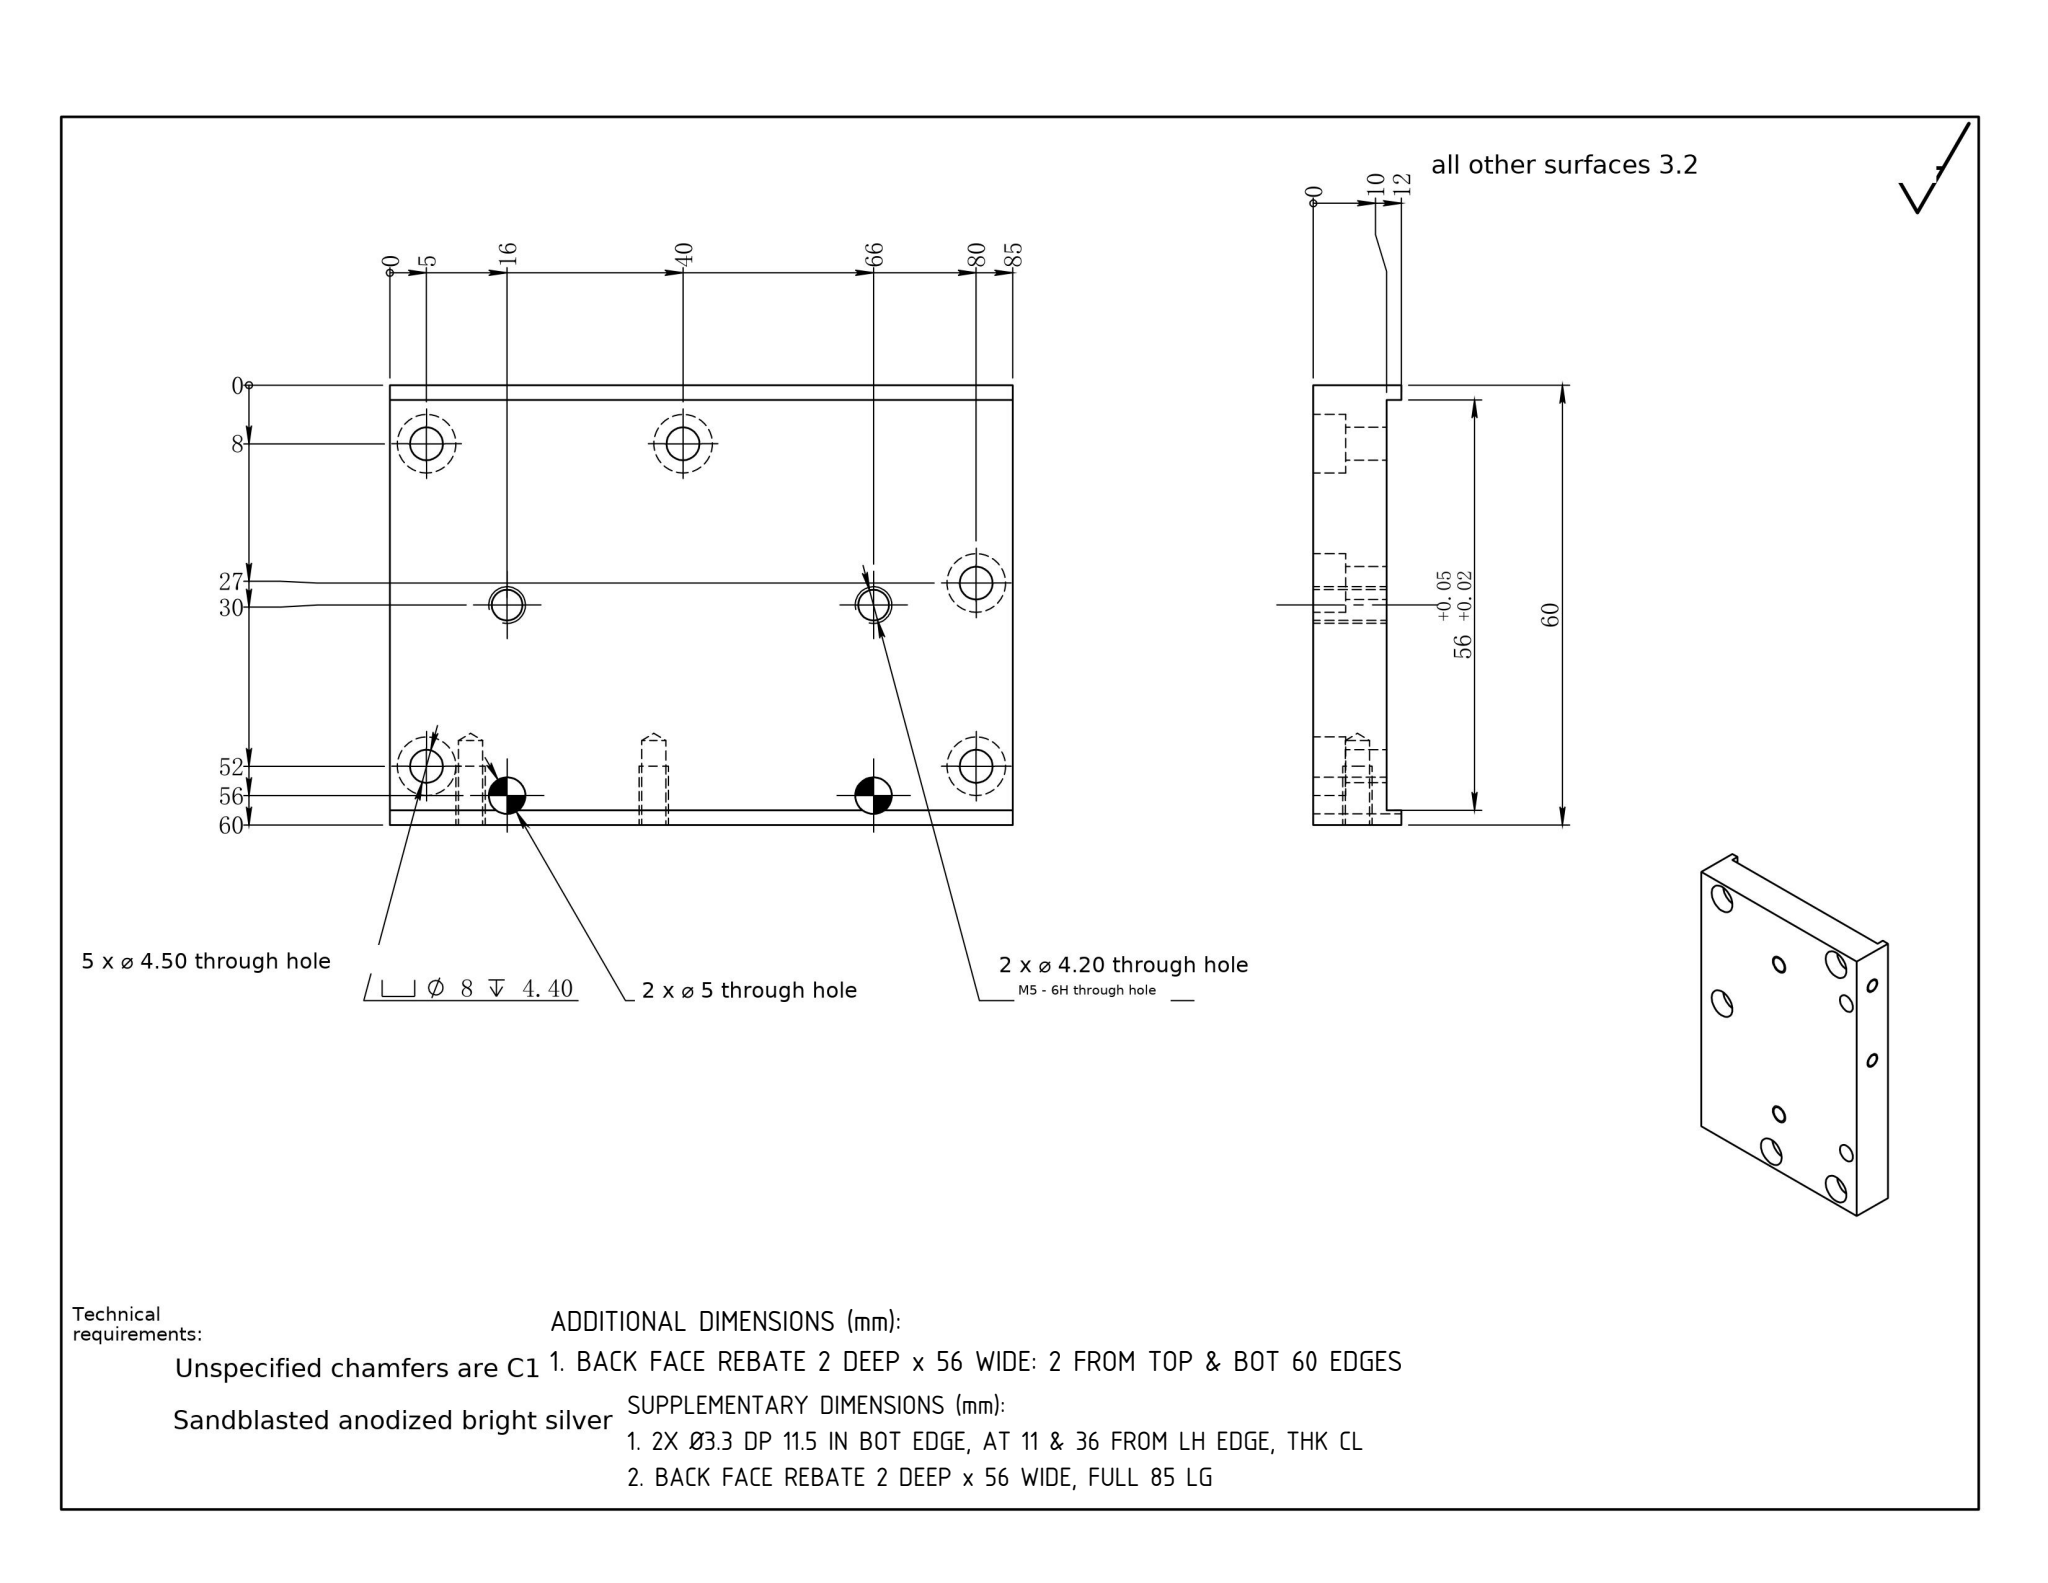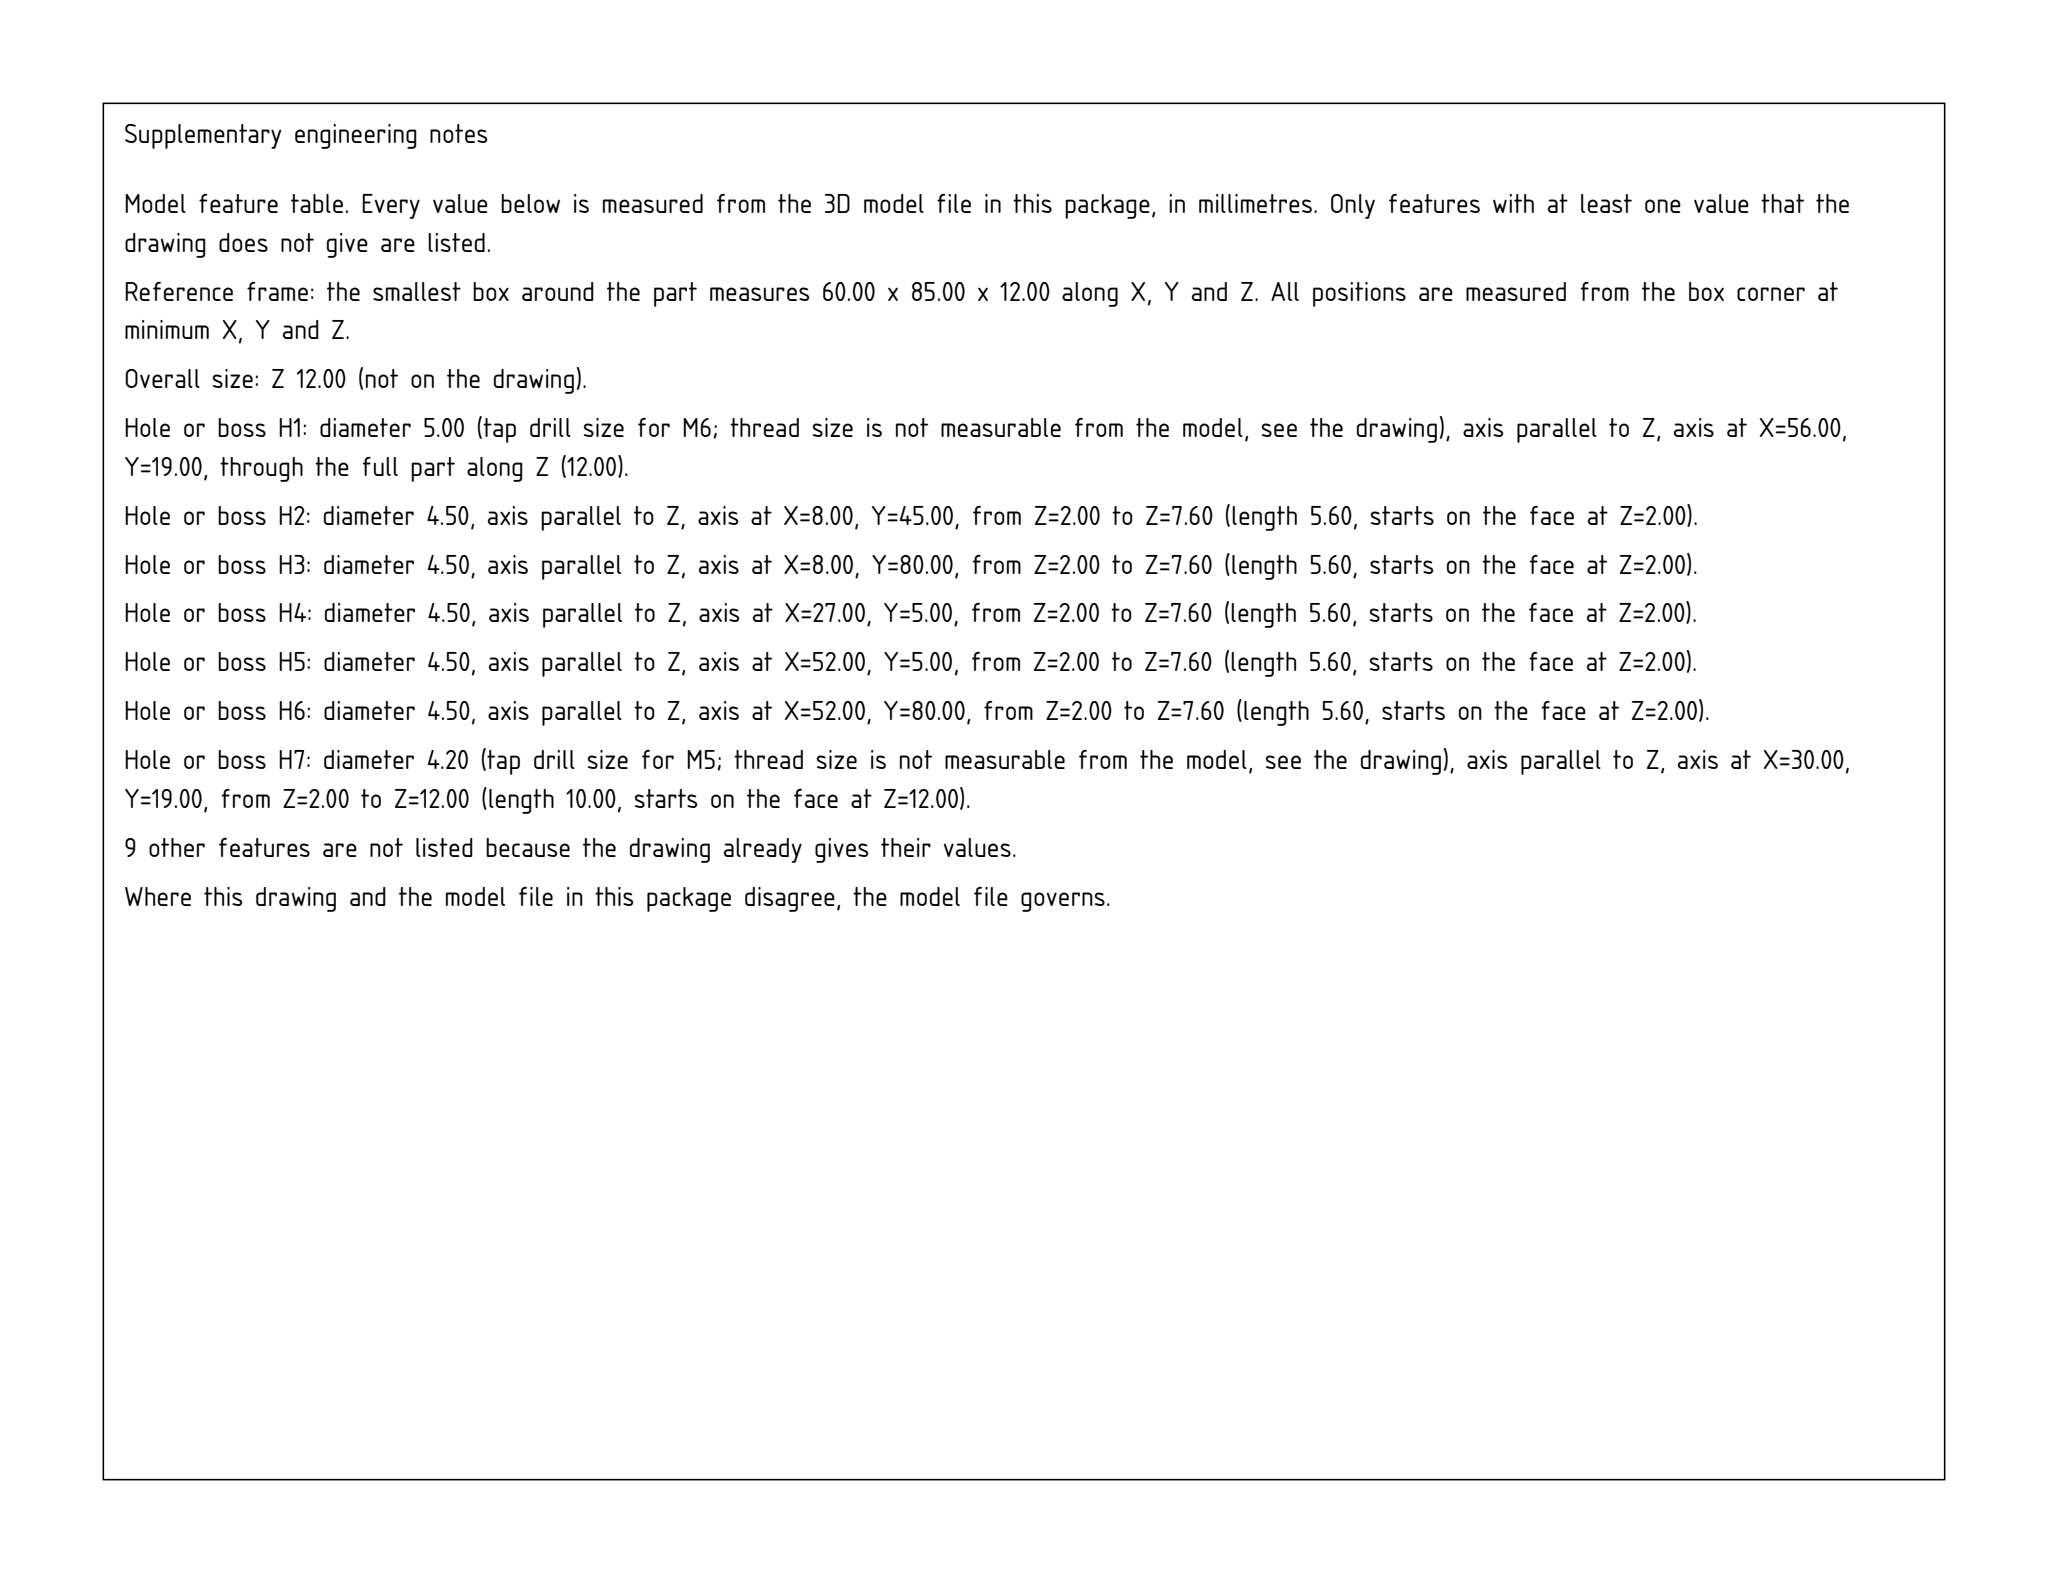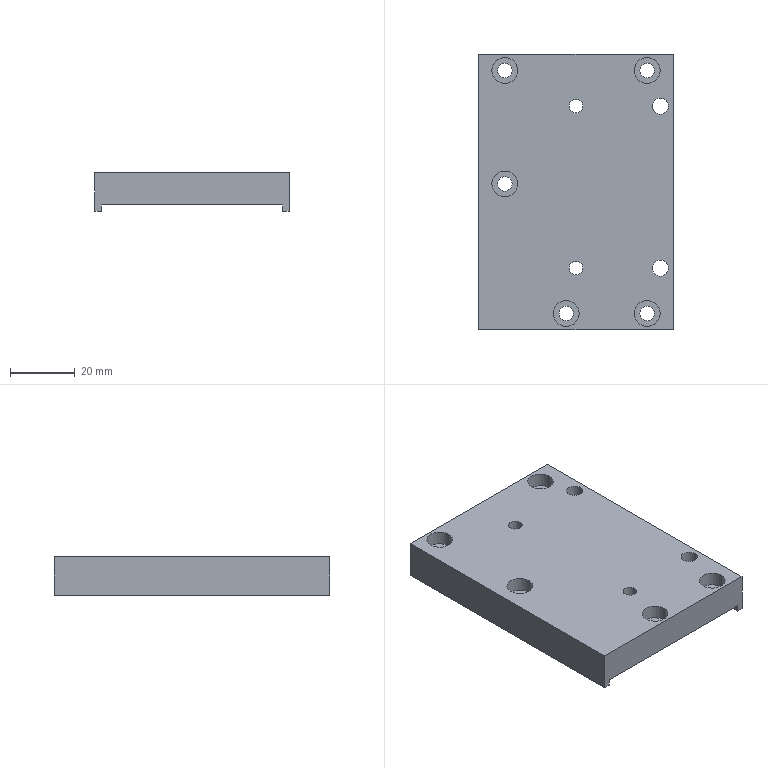Part | SolidWorks | mm | 1 solid | 53 faces | box 60 x 85 x 12 mm | volume 49253 mm3 | cylinder 32 | plane 17 | cone 4 | commonest cylinder face diameters 8 x10 4.5 x10 3.3 x4 5 x4 4.2 x4
build123d program:
from build123d import *

# Parameters (mm, degrees)
SKETCH1_W                                       = 60
SKETCH1_H                                       = 85
BOSS_EXTRUDE1_DEPTH                             = 6
M5_TAPPED_HOLE1_D                               = 4.2
F_5_0_5_DIAMETER_HOLE1_D                        = 5
SKETCH8_W                                       = 56
SKETCH8_H                                       = 85
CUT_EXTRUDE1_DEPTH                              = 2
M4_HEX_SOCKET_HEAD_CAP_SCREW_CBORE1_D           = 4.5
M4_HEX_SOCKET_HEAD_CAP_SCREW_CBORE1_CBORE_D     = 8
M4_HEX_SOCKET_HEAD_CAP_SCREW_CBORE1_CBORE_DEPTH = 4.4
M4_TAPPED_HOLE1_D                               = 3.3
M4_TAPPED_HOLE1_DEPTH                           = 11.5
M4_TAPPED_HOLE1_TIP                             = 0.9914


with BuildPart() as part:
    # Sketch1 → Boss-Extrude1 (new, symmetric)
    with BuildSketch(Plane.XY):
        Rectangle(SKETCH1_W, SKETCH1_H)
    extrude(amount=BOSS_EXTRUDE1_DEPTH, both=True)

    # M5 Tapped Hole1 (through all)
    with Locations(Plane.XY.offset(6)):
        with Locations((0, -23.5), (0, 26.5)):
            Hole(M5_TAPPED_HOLE1_D / 2)

    # 5.0 _5_ Diameter Hole1 (through all)
    with Locations(Plane(origin=(0, 0, -6), x_dir=(-1, 0, 0), z_dir=(0, 0, -1))):
        with Locations((-26, -23.5), (-26, 26.5)):
            Hole(F_5_0_5_DIAMETER_HOLE1_D / 2)

    # Sketch8 → Cut-Extrude1 (cut)
    with BuildSketch(Plane(origin=(0, 0, -6), x_dir=(-1, 0, 0), z_dir=(0, 0, -1))):
        Rectangle(SKETCH8_W, SKETCH8_H)
    extrude(amount=-CUT_EXTRUDE1_DEPTH, mode=Mode.SUBTRACT)

    # M4 Hex Socket Head Cap Screw CBORE1 (through all)
    with Locations(Plane.XY.offset(6)):
        with Locations((-22, 37.5), (22, 37.5), (-22, 2.5), (-3, -37.5), (22, -37.5)):
            CounterBoreHole(M4_HEX_SOCKET_HEAD_CAP_SCREW_CBORE1_D / 2, M4_HEX_SOCKET_HEAD_CAP_SCREW_CBORE1_CBORE_D / 2, M4_HEX_SOCKET_HEAD_CAP_SCREW_CBORE1_CBORE_DEPTH)

    # M4 Tapped Hole1
    with Locations(Plane(origin=(30, 0, 0), x_dir=(0, 0, -1), z_dir=(1, 0, 0))):
        with Locations((0, 31.5), (0, 6.5)):
            Hole(M4_TAPPED_HOLE1_D / 2, depth=M4_TAPPED_HOLE1_DEPTH)
            with Locations((0, 0, -(M4_TAPPED_HOLE1_DEPTH + M4_TAPPED_HOLE1_TIP / 2))):  # 118° drill point
                Cone(0, M4_TAPPED_HOLE1_D / 2, M4_TAPPED_HOLE1_TIP, mode=Mode.SUBTRACT)


solid = part.part